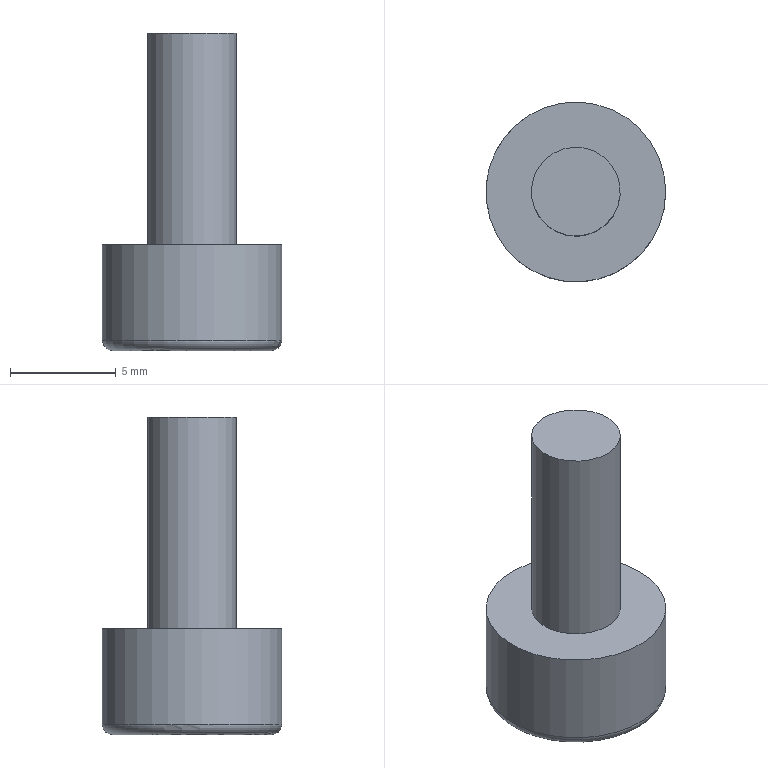Component | NX | 14_T70_1_M5X10_CAP_SCREW | 1 solid | 25 faces | volume 373 mm3 | plane 15 | cone 7 | cylinder 2 | torus 1 | commonest cylinder face diameters 8.5 x1 4.2 x1